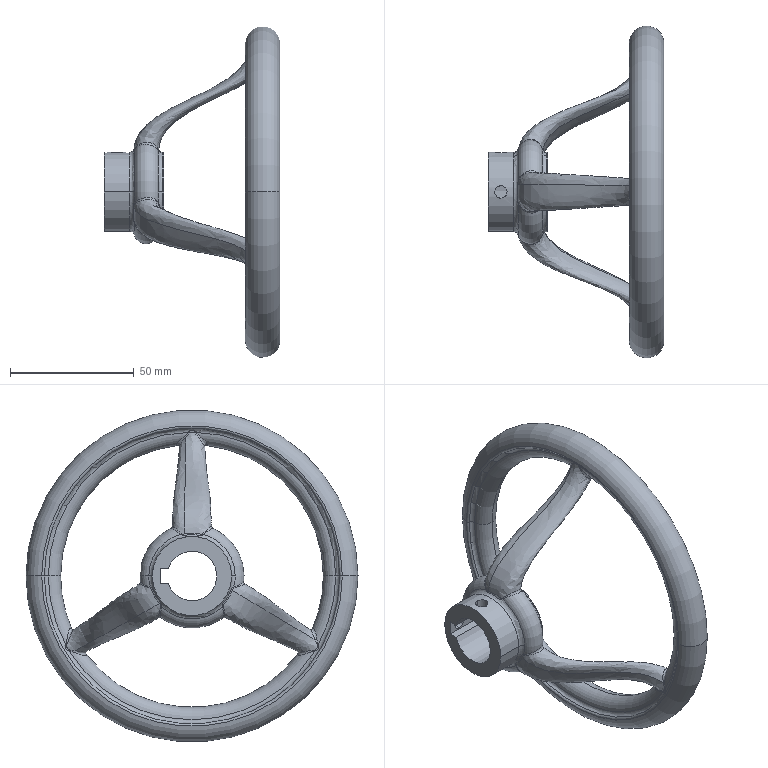Component | SolidWorks | ZL-11-13Handwheel-1 | 1 solid | 63 faces | volume 79509 mm3 | torus 25 | spline 24 | cylinder 9 | plane 5 | commonest cylinder face diameters 5 x4 32 x4 20 x1